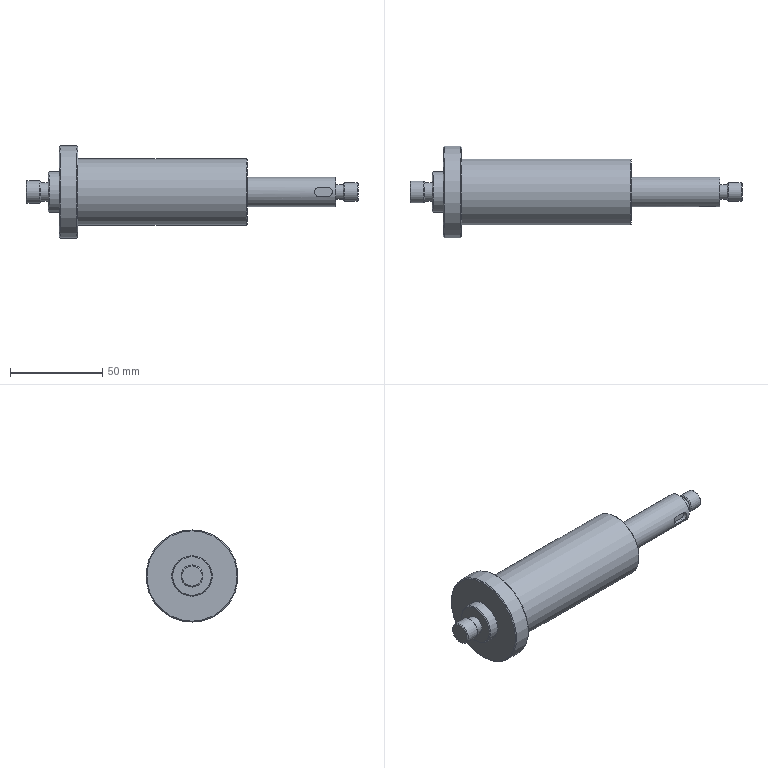Component | NX | SPINDLE | 1 solid | 30 faces | volume 127083 mm3 | plane 12 | cylinder 10 | cone 8 | commonest cylinder face diameters 10 x2 5 x2 8 x1 16 x1 36 x1 50 x1 22 x1 12 x1